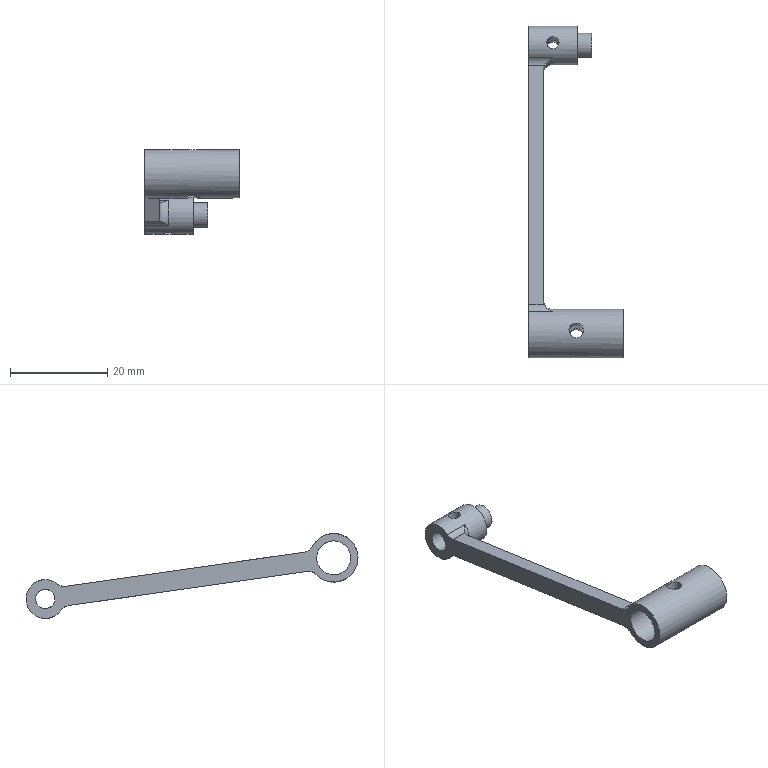Component | NX | 23D__27_2 | 1 solid | 22 faces | volume 1763 mm3 | cylinder 13 | plane 7 | torus 2 | commonest cylinder face diameters 4 x5 2.5 x2 3 x2 10 x1 7 x1 8 x1 5 x1